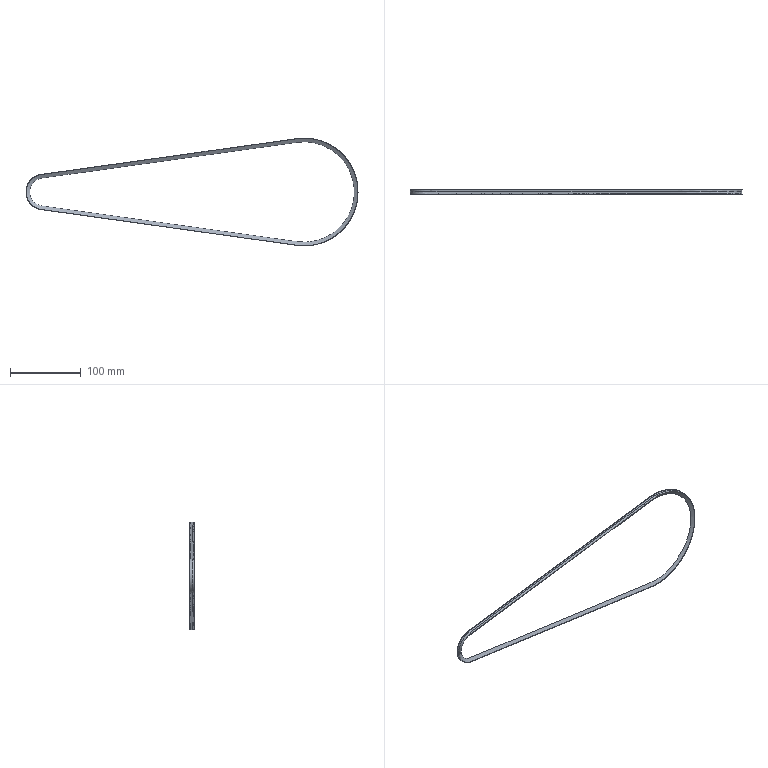Component | NX | LARGE_BELT_4 | 1 solid | 2 faces | volume 18528 mm3 | spline 2